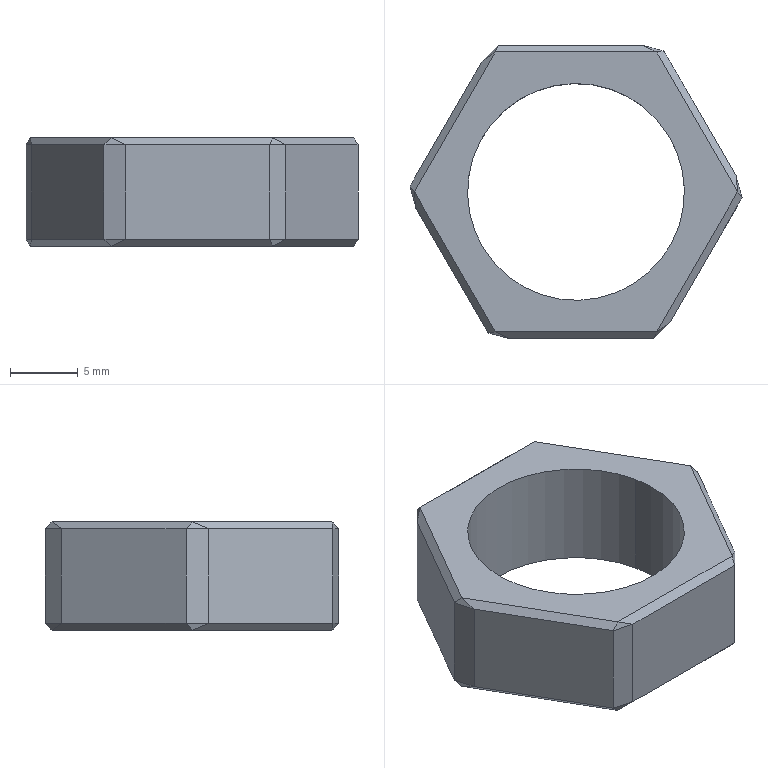Component | SolidWorks | AssemblyVibratoryFeederChassis-1_FootPadScrew-4 | 1 solid | 40 faces | box 24.5 x 21.65 x 8 mm | volume 1608 mm3 | plane 38 | cylinder 2 | commonest cylinder face diameters 16 x2
STEP:
#1=COLOUR_RGB('',0.7922,0.8196,0.9333);
#2=FILL_AREA_STYLE_COLOUR('',#1);
#3=FILL_AREA_STYLE('',(#2));
#4=SURFACE_STYLE_FILL_AREA(#3);
#5=SURFACE_SIDE_STYLE('',(#4));
#6=SURFACE_STYLE_USAGE(.BOTH.,#5);
#7=PRESENTATION_STYLE_ASSIGNMENT((#6));
#8=CARTESIAN_POINT('',(-15.563,9.734,-3.15));
#9=VERTEX_POINT('',#8);
#10=CARTESIAN_POINT('',(-14.945,9.859,-3.15));
#11=VERTEX_POINT('',#10);
#12=CARTESIAN_POINT('',(-15.254,9.796,-3.15));
#13=DIRECTION('',(0.,-0.,1.));
#14=DIRECTION('',(0.98,0.199,0.));
#15=AXIS2_PLACEMENT_3D('',#12,#13,#14);
#16=CIRCLE('',#15,0.315);
#17=EDGE_CURVE('',#9,#11,#16,.T.);
#18=ORIENTED_EDGE('',*,*,#17,.F.);
#19=CARTESIAN_POINT('',(-15.563,9.734,-2.835));
#20=VERTEX_POINT('',#19);
#21=CARTESIAN_POINT('',(-15.563,9.734,-2.835));
#22=DIRECTION('',(0.,-0.,1.));
#23=VECTOR('',#22,39.37);
#24=LINE('',#21,#23);
#25=EDGE_CURVE('',#9,#20,#24,.T.);
#26=ORIENTED_EDGE('',*,*,#25,.T.);
#27=CARTESIAN_POINT('',(-14.945,9.859,-2.835));
#28=VERTEX_POINT('',#27);
#29=CARTESIAN_POINT('',(-15.254,9.796,-2.835));
#30=DIRECTION('',(0.,-0.,1.));
#31=DIRECTION('',(0.98,0.199,0.));
#32=AXIS2_PLACEMENT_3D('',#29,#30,#31);
#33=CIRCLE('',#32,0.315);
#34=EDGE_CURVE('',#20,#28,#33,.T.);
#35=ORIENTED_EDGE('',*,*,#34,.T.);
#36=CARTESIAN_POINT('',(-14.945,9.859,-2.835));
#37=DIRECTION('',(0.,-0.,1.));
#38=VECTOR('',#37,39.37);
#39=LINE('',#36,#38);
#40=EDGE_CURVE('',#11,#28,#39,.T.);
#41=ORIENTED_EDGE('',*,*,#40,.F.);
#42=EDGE_LOOP('',(#18,#26,#35,#41));
#43=FACE_OUTER_BOUND('',#42,.T.);
#44=CARTESIAN_POINT('',(-15.254,9.796,-2.835));
#45=DIRECTION('',(0.,-0.,1.));
#46=DIRECTION('',(0.98,0.199,0.));
#47=AXIS2_PLACEMENT_3D('',#44,#45,#46);
#48=CYLINDRICAL_SURFACE('',#47,0.315);
#49=ADVANCED_FACE('',(#43),#48,.F.);
#50=CARTESIAN_POINT('',(-14.772,9.779,-3.13));
#51=VERTEX_POINT('',#50);
#52=CARTESIAN_POINT('',(-14.772,9.779,-2.854));
#53=VERTEX_POINT('',#52);
#54=CARTESIAN_POINT('',(-14.772,9.779,-2.835));
#55=DIRECTION('',(0.,-0.,1.));
#56=VECTOR('',#55,39.37);
#57=LINE('',#54,#56);
#58=EDGE_CURVE('',#51,#53,#57,.T.);
#59=ORIENTED_EDGE('',*,*,#58,.T.);
#60=CARTESIAN_POINT('',(-14.981,9.417,-2.854));
#61=VERTEX_POINT('',#60);
#62=CARTESIAN_POINT('',(-15.008,9.37,-2.854));
#63=DIRECTION('',(-0.5,-0.866,0.));
#64=VECTOR('',#63,39.37);
#65=LINE('',#62,#64);
#66=EDGE_CURVE('',#53,#61,#65,.T.);
#67=ORIENTED_EDGE('',*,*,#66,.T.);
#68=CARTESIAN_POINT('',(-14.981,9.417,-3.13));
#69=VERTEX_POINT('',#68);
#70=CARTESIAN_POINT('',(-14.981,9.417,-2.835));
#71=DIRECTION('',(-0.,0.,-1.));
#72=VECTOR('',#71,39.37);
#73=LINE('',#70,#72);
#74=EDGE_CURVE('',#61,#69,#73,.T.);
#75=ORIENTED_EDGE('',*,*,#74,.T.);
#76=CARTESIAN_POINT('',(-15.008,9.37,-3.13));
#77=DIRECTION('',(0.5,0.866,-0.));
#78=VECTOR('',#77,39.37);
#79=LINE('',#76,#78);
#80=EDGE_CURVE('',#69,#51,#79,.T.);
#81=ORIENTED_EDGE('',*,*,#80,.T.);
#82=EDGE_LOOP('',(#59,#67,#75,#81));
#83=FACE_OUTER_BOUND('',#82,.T.);
#84=CARTESIAN_POINT('',(-15.008,9.37,-2.835));
#85=DIRECTION('',(-0.866,0.5,0.));
#86=DIRECTION('',(-0.5,-0.866,0.));
#87=AXIS2_PLACEMENT_3D('',#84,#85,#86);
#88=PLANE('',#87);
#89=ADVANCED_FACE('',(#83),#88,.F.);
#90=CARTESIAN_POINT('',(-14.998,10.205,-2.854));
#91=VERTEX_POINT('',#90);
#92=CARTESIAN_POINT('',(-14.789,9.843,-2.854));
#93=VERTEX_POINT('',#92);
#94=CARTESIAN_POINT('',(-14.762,9.796,-2.854));
#95=DIRECTION('',(0.5,-0.866,-0.));
#96=VECTOR('',#95,39.37);
#97=LINE('',#94,#96);
#98=EDGE_CURVE('',#91,#93,#97,.T.);
#99=ORIENTED_EDGE('',*,*,#98,.T.);
#100=CARTESIAN_POINT('',(-14.789,9.843,-3.13));
#101=VERTEX_POINT('',#100);
#102=CARTESIAN_POINT('',(-14.789,9.843,-2.835));
#103=DIRECTION('',(-0.,0.,-1.));
#104=VECTOR('',#103,39.37);
#105=LINE('',#102,#104);
#106=EDGE_CURVE('',#93,#101,#105,.T.);
#107=ORIENTED_EDGE('',*,*,#106,.T.);
#108=CARTESIAN_POINT('',(-14.998,10.205,-3.13));
#109=VERTEX_POINT('',#108);
#110=CARTESIAN_POINT('',(-14.762,9.796,-3.13));
#111=DIRECTION('',(-0.5,0.866,0.));
#112=VECTOR('',#111,39.37);
#113=LINE('',#110,#112);
#114=EDGE_CURVE('',#101,#109,#113,.T.);
#115=ORIENTED_EDGE('',*,*,#114,.T.);
#116=CARTESIAN_POINT('',(-14.998,10.205,-2.835));
#117=DIRECTION('',(0.,-0.,1.));
#118=VECTOR('',#117,39.37);
#119=LINE('',#116,#118);
#120=EDGE_CURVE('',#109,#91,#119,.T.);
#121=ORIENTED_EDGE('',*,*,#120,.T.);
#122=EDGE_LOOP('',(#99,#107,#115,#121));
#123=FACE_OUTER_BOUND('',#122,.T.);
#124=CARTESIAN_POINT('',(-14.762,9.796,-2.835));
#125=DIRECTION('',(-0.866,-0.5,0.));
#126=DIRECTION('',(0.5,-0.866,-0.));
#127=AXIS2_PLACEMENT_3D('',#124,#125,#126);
#128=PLANE('',#127);
#129=ADVANCED_FACE('',(#123),#128,.F.);
#130=CARTESIAN_POINT('',(-15.062,10.222,-3.13));
#131=VERTEX_POINT('',#130);
#132=CARTESIAN_POINT('',(-15.48,10.222,-3.13));
#133=VERTEX_POINT('',#132);
#134=CARTESIAN_POINT('',(-15.008,10.222,-3.13));
#135=DIRECTION('',(-1.,0.,0.));
#136=VECTOR('',#135,39.37);
#137=LINE('',#134,#136);
#138=EDGE_CURVE('',#131,#133,#137,.T.);
#139=ORIENTED_EDGE('',*,*,#138,.T.);
#140=CARTESIAN_POINT('',(-15.48,10.222,-2.854));
#141=VERTEX_POINT('',#140);
#142=CARTESIAN_POINT('',(-15.48,10.222,-2.835));
#143=DIRECTION('',(0.,-0.,1.));
#144=VECTOR('',#143,39.37);
#145=LINE('',#142,#144);
#146=EDGE_CURVE('',#133,#141,#145,.T.);
#147=ORIENTED_EDGE('',*,*,#146,.T.);
#148=CARTESIAN_POINT('',(-15.062,10.222,-2.854));
#149=VERTEX_POINT('',#148);
#150=CARTESIAN_POINT('',(-15.008,10.222,-2.854));
#151=DIRECTION('',(1.,-0.,-0.));
#152=VECTOR('',#151,39.37);
#153=LINE('',#150,#152);
#154=EDGE_CURVE('',#141,#149,#153,.T.);
#155=ORIENTED_EDGE('',*,*,#154,.T.);
#156=CARTESIAN_POINT('',(-15.062,10.222,-2.835));
#157=DIRECTION('',(-0.,0.,-1.));
#158=VECTOR('',#157,39.37);
#159=LINE('',#156,#158);
#160=EDGE_CURVE('',#149,#131,#159,.T.);
#161=ORIENTED_EDGE('',*,*,#160,.T.);
#162=EDGE_LOOP('',(#139,#147,#155,#161));
#163=FACE_OUTER_BOUND('',#162,.T.);
#164=CARTESIAN_POINT('',(-15.008,10.222,-2.835));
#165=DIRECTION('',(-0.,-1.,-0.));
#166=DIRECTION('',(1.,-0.,-0.));
#167=AXIS2_PLACEMENT_3D('',#164,#165,#166);
#168=PLANE('',#167);
#169=ADVANCED_FACE('',(#163),#168,.F.);
#170=CARTESIAN_POINT('',(-15.736,9.813,-3.13));
#171=VERTEX_POINT('',#170);
#172=CARTESIAN_POINT('',(-15.736,9.813,-2.854));
#173=VERTEX_POINT('',#172);
#174=CARTESIAN_POINT('',(-15.736,9.813,-2.835));
#175=DIRECTION('',(0.,-0.,1.));
#176=VECTOR('',#175,39.37);
#177=LINE('',#174,#176);
#178=EDGE_CURVE('',#171,#173,#177,.T.);
#179=ORIENTED_EDGE('',*,*,#178,.T.);
#180=CARTESIAN_POINT('',(-15.527,10.176,-2.854));
#181=VERTEX_POINT('',#180);
#182=CARTESIAN_POINT('',(-15.5,10.222,-2.854));
#183=DIRECTION('',(0.5,0.866,-0.));
#184=VECTOR('',#183,39.37);
#185=LINE('',#182,#184);
#186=EDGE_CURVE('',#173,#181,#185,.T.);
#187=ORIENTED_EDGE('',*,*,#186,.T.);
#188=CARTESIAN_POINT('',(-15.527,10.176,-3.13));
#189=VERTEX_POINT('',#188);
#190=CARTESIAN_POINT('',(-15.527,10.176,-2.835));
#191=DIRECTION('',(-0.,0.,-1.));
#192=VECTOR('',#191,39.37);
#193=LINE('',#190,#192);
#194=EDGE_CURVE('',#181,#189,#193,.T.);
#195=ORIENTED_EDGE('',*,*,#194,.T.);
#196=CARTESIAN_POINT('',(-15.5,10.222,-3.13));
#197=DIRECTION('',(-0.5,-0.866,0.));
#198=VECTOR('',#197,39.37);
#199=LINE('',#196,#198);
#200=EDGE_CURVE('',#189,#171,#199,.T.);
#201=ORIENTED_EDGE('',*,*,#200,.T.);
#202=EDGE_LOOP('',(#179,#187,#195,#201));
#203=FACE_OUTER_BOUND('',#202,.T.);
#204=CARTESIAN_POINT('',(-15.5,10.222,-2.835));
#205=DIRECTION('',(0.866,-0.5,-0.));
#206=DIRECTION('',(0.5,0.866,-0.));
#207=AXIS2_PLACEMENT_3D('',#204,#205,#206);
#208=PLANE('',#207);
#209=ADVANCED_FACE('',(#203),#208,.F.);
#210=CARTESIAN_POINT('',(-15.51,9.387,-3.13));
#211=VERTEX_POINT('',#210);
#212=CARTESIAN_POINT('',(-15.51,9.387,-2.854));
#213=VERTEX_POINT('',#212);
#214=CARTESIAN_POINT('',(-15.51,9.387,-2.835));
#215=DIRECTION('',(0.,-0.,1.));
#216=VECTOR('',#215,39.37);
#217=LINE('',#214,#216);
#218=EDGE_CURVE('',#211,#213,#217,.T.);
#219=ORIENTED_EDGE('',*,*,#218,.T.);
#220=CARTESIAN_POINT('',(-15.719,9.75,-2.854));
#221=VERTEX_POINT('',#220);
#222=CARTESIAN_POINT('',(-15.746,9.796,-2.854));
#223=DIRECTION('',(-0.5,0.866,0.));
#224=VECTOR('',#223,39.37);
#225=LINE('',#222,#224);
#226=EDGE_CURVE('',#213,#221,#225,.T.);
#227=ORIENTED_EDGE('',*,*,#226,.T.);
#228=CARTESIAN_POINT('',(-15.719,9.75,-3.13));
#229=VERTEX_POINT('',#228);
#230=CARTESIAN_POINT('',(-15.719,9.75,-2.835));
#231=DIRECTION('',(-0.,0.,-1.));
#232=VECTOR('',#231,39.37);
#233=LINE('',#230,#232);
#234=EDGE_CURVE('',#221,#229,#233,.T.);
#235=ORIENTED_EDGE('',*,*,#234,.T.);
#236=CARTESIAN_POINT('',(-15.746,9.796,-3.13));
#237=DIRECTION('',(0.5,-0.866,-0.));
#238=VECTOR('',#237,39.37);
#239=LINE('',#236,#238);
#240=EDGE_CURVE('',#229,#211,#239,.T.);
#241=ORIENTED_EDGE('',*,*,#240,.T.);
#242=EDGE_LOOP('',(#219,#227,#235,#241));
#243=FACE_OUTER_BOUND('',#242,.T.);
#244=CARTESIAN_POINT('',(-15.746,9.796,-2.835));
#245=DIRECTION('',(0.866,0.5,-0.));
#246=DIRECTION('',(-0.5,0.866,0.));
#247=AXIS2_PLACEMENT_3D('',#244,#245,#246);
#248=PLANE('',#247);
#249=ADVANCED_FACE('',(#243),#248,.F.);
#250=CARTESIAN_POINT('',(-15.028,9.37,-3.13));
#251=VERTEX_POINT('',#250);
#252=CARTESIAN_POINT('',(-15.028,9.37,-2.854));
#253=VERTEX_POINT('',#252);
#254=CARTESIAN_POINT('',(-15.028,9.37,-2.835));
#255=DIRECTION('',(0.,-0.,1.));
#256=VECTOR('',#255,39.37);
#257=LINE('',#254,#256);
#258=EDGE_CURVE('',#251,#253,#257,.T.);
#259=ORIENTED_EDGE('',*,*,#258,.T.);
#260=CARTESIAN_POINT('',(-15.446,9.37,-2.854));
#261=VERTEX_POINT('',#260);
#262=CARTESIAN_POINT('',(-15.5,9.37,-2.854));
#263=DIRECTION('',(-1.,0.,0.));
#264=VECTOR('',#263,39.37);
#265=LINE('',#262,#264);
#266=EDGE_CURVE('',#253,#261,#265,.T.);
#267=ORIENTED_EDGE('',*,*,#266,.T.);
#268=CARTESIAN_POINT('',(-15.446,9.37,-3.13));
#269=VERTEX_POINT('',#268);
#270=CARTESIAN_POINT('',(-15.446,9.37,-2.835));
#271=DIRECTION('',(-0.,0.,-1.));
#272=VECTOR('',#271,39.37);
#273=LINE('',#270,#272);
#274=EDGE_CURVE('',#261,#269,#273,.T.);
#275=ORIENTED_EDGE('',*,*,#274,.T.);
#276=CARTESIAN_POINT('',(-15.5,9.37,-3.13));
#277=DIRECTION('',(1.,-0.,-0.));
#278=VECTOR('',#277,39.37);
#279=LINE('',#276,#278);
#280=EDGE_CURVE('',#269,#251,#279,.T.);
#281=ORIENTED_EDGE('',*,*,#280,.T.);
#282=EDGE_LOOP('',(#259,#267,#275,#281));
#283=FACE_OUTER_BOUND('',#282,.T.);
#284=CARTESIAN_POINT('',(-15.5,9.37,-2.835));
#285=DIRECTION('',(0.,1.,0.));
#286=DIRECTION('',(-1.,0.,0.));
#287=AXIS2_PLACEMENT_3D('',#284,#285,#286);
#288=PLANE('',#287);
#289=ADVANCED_FACE('',(#283),#288,.F.);
#290=CARTESIAN_POINT('',(-15.489,9.39,-2.835));
#291=VERTEX_POINT('',#290);
#292=CARTESIAN_POINT('',(-15.019,9.39,-2.835));
#293=VERTEX_POINT('',#292);
#294=CARTESIAN_POINT('',(-15.008,9.39,-2.835));
#295=DIRECTION('',(1.,-0.,-0.));
#296=VECTOR('',#295,39.37);
#297=LINE('',#294,#296);
#298=EDGE_CURVE('',#291,#293,#297,.T.);
#299=ORIENTED_EDGE('',*,*,#298,.T.);
#300=CARTESIAN_POINT('',(-14.784,9.796,-2.835));
#301=VERTEX_POINT('',#300);
#302=CARTESIAN_POINT('',(-14.779,9.806,-2.835));
#303=DIRECTION('',(0.5,0.866,-0.));
#304=VECTOR('',#303,39.37);
#305=LINE('',#302,#304);
#306=EDGE_CURVE('',#293,#301,#305,.T.);
#307=ORIENTED_EDGE('',*,*,#306,.T.);
#308=CARTESIAN_POINT('',(-15.019,10.203,-2.835));
#309=VERTEX_POINT('',#308);
#310=CARTESIAN_POINT('',(-15.025,10.213,-2.835));
#311=DIRECTION('',(-0.5,0.866,0.));
#312=VECTOR('',#311,39.37);
#313=LINE('',#310,#312);
#314=EDGE_CURVE('',#301,#309,#313,.T.);
#315=ORIENTED_EDGE('',*,*,#314,.T.);
#316=CARTESIAN_POINT('',(-15.489,10.203,-2.835));
#317=VERTEX_POINT('',#316);
#318=CARTESIAN_POINT('',(-15.5,10.203,-2.835));
#319=DIRECTION('',(-1.,0.,0.));
#320=VECTOR('',#319,39.37);
#321=LINE('',#318,#320);
#322=EDGE_CURVE('',#309,#317,#321,.T.);
#323=ORIENTED_EDGE('',*,*,#322,.T.);
#324=CARTESIAN_POINT('',(-15.723,9.796,-2.835));
#325=VERTEX_POINT('',#324);
#326=CARTESIAN_POINT('',(-15.729,9.786,-2.835));
#327=DIRECTION('',(-0.5,-0.866,0.));
#328=VECTOR('',#327,39.37);
#329=LINE('',#326,#328);
#330=EDGE_CURVE('',#317,#325,#329,.T.);
#331=ORIENTED_EDGE('',*,*,#330,.T.);
#332=CARTESIAN_POINT('',(-15.483,9.38,-2.835));
#333=DIRECTION('',(0.5,-0.866,-0.));
#334=VECTOR('',#333,39.37);
#335=LINE('',#332,#334);
#336=EDGE_CURVE('',#325,#291,#335,.T.);
#337=ORIENTED_EDGE('',*,*,#336,.T.);
#338=EDGE_LOOP('',(#299,#307,#315,#323,#331,#337));
#339=FACE_OUTER_BOUND('',#338,.T.);
#340=CARTESIAN_POINT('',(-15.254,9.796,-2.835));
#341=DIRECTION('',(0.,-0.,1.));
#342=DIRECTION('',(0.98,0.199,0.));
#343=AXIS2_PLACEMENT_3D('',#340,#341,#342);
#344=CIRCLE('',#343,0.315);
#345=EDGE_CURVE('',#28,#20,#344,.T.);
#346=ORIENTED_EDGE('',*,*,#345,.F.);
#347=ORIENTED_EDGE('',*,*,#34,.F.);
#348=EDGE_LOOP('',(#346,#347));
#349=FACE_BOUND('',#348,.T.);
#350=CARTESIAN_POINT('',(-14.762,9.796,-2.835));
#351=DIRECTION('',(0.,-0.,1.));
#352=DIRECTION('',(0.98,0.199,-0.));
#353=AXIS2_PLACEMENT_3D('',#350,#351,#352);
#354=PLANE('',#353);
#355=ADVANCED_FACE('',(#339,#349),#354,.T.);
#356=CARTESIAN_POINT('',(-15.019,10.203,-3.15));
#357=VERTEX_POINT('',#356);
#358=CARTESIAN_POINT('',(-14.784,9.796,-3.15));
#359=VERTEX_POINT('',#358);
#360=CARTESIAN_POINT('',(-14.779,9.786,-3.15));
#361=DIRECTION('',(0.5,-0.866,-0.));
#362=VECTOR('',#361,39.37);
#363=LINE('',#360,#362);
#364=EDGE_CURVE('',#357,#359,#363,.T.);
#365=ORIENTED_EDGE('',*,*,#364,.T.);
#366=CARTESIAN_POINT('',(-15.019,9.39,-3.15));
#367=VERTEX_POINT('',#366);
#368=CARTESIAN_POINT('',(-14.779,9.806,-3.15));
#369=DIRECTION('',(-0.5,-0.866,0.));
#370=VECTOR('',#369,39.37);
#371=LINE('',#368,#370);
#372=EDGE_CURVE('',#359,#367,#371,.T.);
#373=ORIENTED_EDGE('',*,*,#372,.T.);
#374=CARTESIAN_POINT('',(-15.489,9.39,-3.15));
#375=VERTEX_POINT('',#374);
#376=CARTESIAN_POINT('',(-14.762,9.39,-3.15));
#377=DIRECTION('',(-1.,0.,0.));
#378=VECTOR('',#377,39.37);
#379=LINE('',#376,#378);
#380=EDGE_CURVE('',#367,#375,#379,.T.);
#381=ORIENTED_EDGE('',*,*,#380,.T.);
#382=CARTESIAN_POINT('',(-15.723,9.796,-3.15));
#383=VERTEX_POINT('',#382);
#384=CARTESIAN_POINT('',(-15.483,9.38,-3.15));
#385=DIRECTION('',(-0.5,0.866,0.));
#386=VECTOR('',#385,39.37);
#387=LINE('',#384,#386);
#388=EDGE_CURVE('',#375,#383,#387,.T.);
#389=ORIENTED_EDGE('',*,*,#388,.T.);
#390=CARTESIAN_POINT('',(-15.489,10.203,-3.15));
#391=VERTEX_POINT('',#390);
#392=CARTESIAN_POINT('',(-15.483,10.213,-3.15));
#393=DIRECTION('',(0.5,0.866,-0.));
#394=VECTOR('',#393,39.37);
#395=LINE('',#392,#394);
#396=EDGE_CURVE('',#383,#391,#395,.T.);
#397=ORIENTED_EDGE('',*,*,#396,.T.);
#398=CARTESIAN_POINT('',(-14.762,10.203,-3.15));
#399=DIRECTION('',(1.,-0.,-0.));
#400=VECTOR('',#399,39.37);
#401=LINE('',#398,#400);
#402=EDGE_CURVE('',#391,#357,#401,.T.);
#403=ORIENTED_EDGE('',*,*,#402,.T.);
#404=EDGE_LOOP('',(#365,#373,#381,#389,#397,#403));
#405=FACE_OUTER_BOUND('',#404,.T.);
#406=CARTESIAN_POINT('',(-15.254,9.796,-3.15));
#407=DIRECTION('',(0.,-0.,1.));
#408=DIRECTION('',(0.98,0.199,0.));
#409=AXIS2_PLACEMENT_3D('',#406,#407,#408);
#410=CIRCLE('',#409,0.315);
#411=EDGE_CURVE('',#11,#9,#410,.T.);
#412=ORIENTED_EDGE('',*,*,#411,.T.);
#413=ORIENTED_EDGE('',*,*,#17,.T.);
#414=EDGE_LOOP('',(#412,#413));
#415=FACE_BOUND('',#414,.T.);
#416=CARTESIAN_POINT('',(-14.762,9.796,-3.15));
#417=DIRECTION('',(0.,-0.,1.));
#418=DIRECTION('',(0.98,0.199,-0.));
#419=AXIS2_PLACEMENT_3D('',#416,#417,#418);
#420=PLANE('',#419);
#421=ADVANCED_FACE('',(#405,#415),#420,.F.);
#422=ORIENTED_EDGE('',*,*,#25,.F.);
#423=ORIENTED_EDGE('',*,*,#411,.F.);
#424=ORIENTED_EDGE('',*,*,#40,.T.);
#425=ORIENTED_EDGE('',*,*,#345,.T.);
#426=EDGE_LOOP('',(#422,#423,#424,#425));
#427=FACE_OUTER_BOUND('',#426,.T.);
#428=CARTESIAN_POINT('',(-15.254,9.796,-2.835));
#429=DIRECTION('',(0.,-0.,1.));
#430=DIRECTION('',(0.98,0.199,0.));
#431=AXIS2_PLACEMENT_3D('',#428,#429,#430);
#432=CYLINDRICAL_SURFACE('',#431,0.315);
#433=ADVANCED_FACE('',(#427),#432,.F.);
#434=CARTESIAN_POINT('',(-15.48,10.222,-2.854));
#435=DIRECTION('',(-0.7071,-0.7071,0.));
#436=VECTOR('',#435,39.37);
#437=LINE('',#434,#436);
#438=EDGE_CURVE('',#141,#181,#437,.T.);
#439=ORIENTED_EDGE('',*,*,#438,.F.);
#440=ORIENTED_EDGE('',*,*,#146,.F.);
#441=CARTESIAN_POINT('',(-15.527,10.176,-3.13));
#442=DIRECTION('',(0.7071,0.7071,0.));
#443=VECTOR('',#442,39.37);
#444=LINE('',#441,#443);
#445=EDGE_CURVE('',#189,#133,#444,.T.);
#446=ORIENTED_EDGE('',*,*,#445,.F.);
#447=ORIENTED_EDGE('',*,*,#194,.F.);
#448=EDGE_LOOP('',(#439,#440,#446,#447));
#449=FACE_OUTER_BOUND('',#448,.T.);
#450=CARTESIAN_POINT('',(-15.527,10.176,-2.835));
#451=DIRECTION('',(0.7071,-0.7071,-0.));
#452=DIRECTION('',(0.7071,0.7071,-0.));
#453=AXIS2_PLACEMENT_3D('',#450,#451,#452);
#454=PLANE('',#453);
#455=ADVANCED_FACE('',(#449),#454,.F.);
#456=CARTESIAN_POINT('',(-15.48,10.222,-2.854));
#457=DIRECTION('',(-0.2863,-0.6775,0.6775));
#458=VECTOR('',#457,39.37);
#459=LINE('',#456,#458);
#460=EDGE_CURVE('',#141,#317,#459,.T.);
#461=ORIENTED_EDGE('',*,*,#460,.F.);
#462=ORIENTED_EDGE('',*,*,#438,.T.);
#463=CARTESIAN_POINT('',(-15.482,10.208,-2.831));
#464=DIRECTION('',(-0.754,-0.53,-0.388));
#465=VECTOR('',#464,39.37);
#466=LINE('',#463,#465);
#467=EDGE_CURVE('',#317,#181,#466,.T.);
#468=ORIENTED_EDGE('',*,*,#467,.F.);
#469=EDGE_LOOP('',(#461,#462,#468));
#470=FACE_OUTER_BOUND('',#469,.T.);
#471=CARTESIAN_POINT('',(-15.48,10.222,-2.854));
#472=DIRECTION('',(-0.6547,0.6547,0.378));
#473=DIRECTION('',(-0.7071,-0.7071,0.));
#474=AXIS2_PLACEMENT_3D('',#471,#472,#473);
#475=PLANE('',#474);
#476=ADVANCED_FACE('',(#470),#475,.T.);
#477=CARTESIAN_POINT('',(-15.527,10.176,-3.13));
#478=DIRECTION('',(0.754,0.53,-0.388));
#479=VECTOR('',#478,39.37);
#480=LINE('',#477,#479);
#481=EDGE_CURVE('',#189,#391,#480,.T.);
#482=ORIENTED_EDGE('',*,*,#481,.F.);
#483=ORIENTED_EDGE('',*,*,#445,.T.);
#484=CARTESIAN_POINT('',(-15.493,10.192,-3.16));
#485=DIRECTION('',(0.2863,0.6775,0.6775));
#486=VECTOR('',#485,39.37);
#487=LINE('',#484,#486);
#488=EDGE_CURVE('',#391,#133,#487,.T.);
#489=ORIENTED_EDGE('',*,*,#488,.F.);
#490=EDGE_LOOP('',(#482,#483,#489));
#491=FACE_OUTER_BOUND('',#490,.T.);
#492=CARTESIAN_POINT('',(-15.527,10.176,-3.13));
#493=DIRECTION('',(-0.6547,0.6547,-0.378));
#494=DIRECTION('',(-0.7071,-0.7071,0.));
#495=AXIS2_PLACEMENT_3D('',#492,#493,#494);
#496=PLANE('',#495);
#497=ADVANCED_FACE('',(#491),#496,.T.);
#498=ORIENTED_EDGE('',*,*,#467,.T.);
#499=ORIENTED_EDGE('',*,*,#186,.F.);
#500=CARTESIAN_POINT('',(-15.736,9.813,-2.854));
#501=DIRECTION('',(-0.4436,0.5867,-0.6775));
#502=VECTOR('',#501,39.37);
#503=LINE('',#500,#502);
#504=EDGE_CURVE('',#325,#173,#503,.T.);
#505=ORIENTED_EDGE('',*,*,#504,.F.);
#506=ORIENTED_EDGE('',*,*,#330,.F.);
#507=EDGE_LOOP('',(#498,#499,#505,#506));
#508=FACE_OUTER_BOUND('',#507,.T.);
#509=CARTESIAN_POINT('',(-15.483,10.213,-2.835));
#510=DIRECTION('',(-0.6124,0.3536,0.7071));
#511=DIRECTION('',(0.7843,0.1593,0.5996));
#512=AXIS2_PLACEMENT_3D('',#509,#510,#511);
#513=PLANE('',#512);
#514=ADVANCED_FACE('',(#508),#513,.T.);
#515=ORIENTED_EDGE('',*,*,#460,.T.);
#516=ORIENTED_EDGE('',*,*,#322,.F.);
#517=CARTESIAN_POINT('',(-15.062,10.222,-2.854));
#518=DIRECTION('',(0.836,-0.388,0.388));
#519=VECTOR('',#518,39.37);
#520=LINE('',#517,#519);
#521=EDGE_CURVE('',#149,#309,#520,.T.);
#522=ORIENTED_EDGE('',*,*,#521,.F.);
#523=ORIENTED_EDGE('',*,*,#154,.F.);
#524=EDGE_LOOP('',(#515,#516,#522,#523));
#525=FACE_OUTER_BOUND('',#524,.T.);
#526=CARTESIAN_POINT('',(-14.762,10.203,-2.835));
#527=DIRECTION('',(0.,0.7071,0.7071));
#528=DIRECTION('',(0.1422,-0.6999,0.6999));
#529=AXIS2_PLACEMENT_3D('',#526,#527,#528);
#530=PLANE('',#529);
#531=ADVANCED_FACE('',(#525),#530,.T.);
#532=CARTESIAN_POINT('',(-15.062,10.222,-3.13));
#533=DIRECTION('',(0.9659,-0.2588,0.));
#534=VECTOR('',#533,39.37);
#535=LINE('',#532,#534);
#536=EDGE_CURVE('',#131,#109,#535,.T.);
#537=ORIENTED_EDGE('',*,*,#536,.F.);
#538=ORIENTED_EDGE('',*,*,#160,.F.);
#539=CARTESIAN_POINT('',(-15.062,10.222,-2.854));
#540=DIRECTION('',(-0.9659,0.2588,0.));
#541=VECTOR('',#540,39.37);
#542=LINE('',#539,#541);
#543=EDGE_CURVE('',#91,#149,#542,.T.);
#544=ORIENTED_EDGE('',*,*,#543,.F.);
#545=ORIENTED_EDGE('',*,*,#120,.F.);
#546=EDGE_LOOP('',(#537,#538,#544,#545));
#547=FACE_OUTER_BOUND('',#546,.T.);
#548=CARTESIAN_POINT('',(-15.062,10.222,-2.835));
#549=DIRECTION('',(-0.2588,-0.9659,-0.));
#550=DIRECTION('',(0.9659,-0.2588,-0.));
#551=AXIS2_PLACEMENT_3D('',#548,#549,#550);
#552=PLANE('',#551);
#553=ADVANCED_FACE('',(#547),#552,.F.);
#554=ORIENTED_EDGE('',*,*,#488,.T.);
#555=ORIENTED_EDGE('',*,*,#138,.F.);
#556=CARTESIAN_POINT('',(-15.062,10.222,-3.13));
#557=DIRECTION('',(-0.836,0.388,0.388));
#558=VECTOR('',#557,39.37);
#559=LINE('',#556,#558);
#560=EDGE_CURVE('',#357,#131,#559,.T.);
#561=ORIENTED_EDGE('',*,*,#560,.F.);
#562=ORIENTED_EDGE('',*,*,#402,.F.);
#563=EDGE_LOOP('',(#554,#555,#561,#562));
#564=FACE_OUTER_BOUND('',#563,.T.);
#565=CARTESIAN_POINT('',(-15.008,10.222,-3.13));
#566=DIRECTION('',(-0.,-0.7071,0.7071));
#567=DIRECTION('',(0.1422,-0.6999,-0.6999));
#568=AXIS2_PLACEMENT_3D('',#565,#566,#567);
#569=PLANE('',#568);
#570=ADVANCED_FACE('',(#564),#569,.F.);
#571=ORIENTED_EDGE('',*,*,#481,.T.);
#572=ORIENTED_EDGE('',*,*,#396,.F.);
#573=CARTESIAN_POINT('',(-15.716,9.787,-3.16));
#574=DIRECTION('',(0.4436,-0.5867,-0.6775));
#575=VECTOR('',#574,39.37);
#576=LINE('',#573,#575);
#577=EDGE_CURVE('',#171,#383,#576,.T.);
#578=ORIENTED_EDGE('',*,*,#577,.F.);
#579=ORIENTED_EDGE('',*,*,#200,.F.);
#580=EDGE_LOOP('',(#571,#572,#578,#579));
#581=FACE_OUTER_BOUND('',#580,.T.);
#582=CARTESIAN_POINT('',(-15.5,10.222,-3.13));
#583=DIRECTION('',(0.6124,-0.3536,0.7071));
#584=DIRECTION('',(0.7843,0.1593,-0.5996));
#585=AXIS2_PLACEMENT_3D('',#582,#583,#584);
#586=PLANE('',#585);
#587=ADVANCED_FACE('',(#581),#586,.F.);
#588=CARTESIAN_POINT('',(-15.736,9.813,-2.854));
#589=DIRECTION('',(0.2588,-0.9659,0.));
#590=VECTOR('',#589,39.37);
#591=LINE('',#588,#590);
#592=EDGE_CURVE('',#173,#221,#591,.T.);
#593=ORIENTED_EDGE('',*,*,#592,.F.);
#594=ORIENTED_EDGE('',*,*,#178,.F.);
#595=CARTESIAN_POINT('',(-15.719,9.75,-3.13));
#596=DIRECTION('',(-0.2588,0.9659,-0.));
#597=VECTOR('',#596,39.37);
#598=LINE('',#595,#597);
#599=EDGE_CURVE('',#229,#171,#598,.T.);
#600=ORIENTED_EDGE('',*,*,#599,.F.);
#601=ORIENTED_EDGE('',*,*,#234,.F.);
#602=EDGE_LOOP('',(#593,#594,#600,#601));
#603=FACE_OUTER_BOUND('',#602,.T.);
#604=CARTESIAN_POINT('',(-15.719,9.75,-2.835));
#605=DIRECTION('',(0.9659,0.2588,-0.));
#606=DIRECTION('',(-0.2588,0.9659,0.));
#607=AXIS2_PLACEMENT_3D('',#604,#605,#606);
#608=PLANE('',#607);
#609=ADVANCED_FACE('',(#603),#608,.F.);
#610=ORIENTED_EDGE('',*,*,#504,.T.);
#611=ORIENTED_EDGE('',*,*,#592,.T.);
#612=CARTESIAN_POINT('',(-15.724,9.805,-2.831));
#613=DIRECTION('',(0.08199,-0.918,-0.388));
#614=VECTOR('',#613,39.37);
#615=LINE('',#612,#614);
#616=EDGE_CURVE('',#325,#221,#615,.T.);
#617=ORIENTED_EDGE('',*,*,#616,.F.);
#618=EDGE_LOOP('',(#610,#611,#617));
#619=FACE_OUTER_BOUND('',#618,.T.);
#620=CARTESIAN_POINT('',(-15.736,9.813,-2.854));
#621=DIRECTION('',(-0.8943,-0.2396,0.378));
#622=DIRECTION('',(0.371,0.07535,0.9256));
#623=AXIS2_PLACEMENT_3D('',#620,#621,#622);
#624=PLANE('',#623);
#625=ADVANCED_FACE('',(#619),#624,.T.);
#626=ORIENTED_EDGE('',*,*,#543,.T.);
#627=ORIENTED_EDGE('',*,*,#521,.T.);
#628=CARTESIAN_POINT('',(-15.031,10.201,-2.824));
#629=DIRECTION('',(-0.7299,-0.09077,0.6775));
#630=VECTOR('',#629,39.37);
#631=LINE('',#628,#630);
#632=EDGE_CURVE('',#91,#309,#631,.T.);
#633=ORIENTED_EDGE('',*,*,#632,.F.);
#634=EDGE_LOOP('',(#626,#627,#633));
#635=FACE_OUTER_BOUND('',#634,.T.);
#636=CARTESIAN_POINT('',(-15.062,10.222,-2.854));
#637=DIRECTION('',(0.2396,0.8943,0.378));
#638=DIRECTION('',(-0.9659,0.2588,0.));
#639=AXIS2_PLACEMENT_3D('',#636,#637,#638);
#640=PLANE('',#639);
#641=ADVANCED_FACE('',(#635),#640,.T.);
#642=ORIENTED_EDGE('',*,*,#560,.T.);
#643=ORIENTED_EDGE('',*,*,#536,.T.);
#644=CARTESIAN_POINT('',(-15.031,10.201,-3.16));
#645=DIRECTION('',(0.7299,0.09077,0.6775));
#646=VECTOR('',#645,39.37);
#647=LINE('',#644,#646);
#648=EDGE_CURVE('',#357,#109,#647,.T.);
#649=ORIENTED_EDGE('',*,*,#648,.F.);
#650=EDGE_LOOP('',(#642,#643,#649));
#651=FACE_OUTER_BOUND('',#650,.T.);
#652=CARTESIAN_POINT('',(-15.062,10.222,-3.13));
#653=DIRECTION('',(0.2396,0.8943,-0.378));
#654=DIRECTION('',(-0.9659,0.2588,0.));
#655=AXIS2_PLACEMENT_3D('',#652,#653,#654);
#656=PLANE('',#655);
#657=ADVANCED_FACE('',(#651),#656,.T.);
#658=ORIENTED_EDGE('',*,*,#599,.T.);
#659=ORIENTED_EDGE('',*,*,#577,.T.);
#660=CARTESIAN_POINT('',(-15.719,9.75,-3.13));
#661=DIRECTION('',(-0.08199,0.918,-0.388));
#662=VECTOR('',#661,39.37);
#663=LINE('',#660,#662);
#664=EDGE_CURVE('',#229,#383,#663,.T.);
#665=ORIENTED_EDGE('',*,*,#664,.F.);
#666=EDGE_LOOP('',(#658,#659,#665));
#667=FACE_OUTER_BOUND('',#666,.T.);
#668=CARTESIAN_POINT('',(-15.719,9.75,-3.13));
#669=DIRECTION('',(-0.8943,-0.2396,-0.378));
#670=DIRECTION('',(-0.371,-0.07535,0.9256));
#671=AXIS2_PLACEMENT_3D('',#668,#669,#670);
#672=PLANE('',#671);
#673=ADVANCED_FACE('',(#667),#672,.T.);
#674=ORIENTED_EDGE('',*,*,#616,.T.);
#675=ORIENTED_EDGE('',*,*,#226,.F.);
#676=CARTESIAN_POINT('',(-15.51,9.387,-2.854));
#677=DIRECTION('',(-0.7299,-0.09077,-0.6775));
#678=VECTOR('',#677,39.37);
#679=LINE('',#676,#678);
#680=EDGE_CURVE('',#291,#213,#679,.T.);
#681=ORIENTED_EDGE('',*,*,#680,.F.);
#682=ORIENTED_EDGE('',*,*,#336,.F.);
#683=EDGE_LOOP('',(#674,#675,#681,#682));
#684=FACE_OUTER_BOUND('',#683,.T.);
#685=CARTESIAN_POINT('',(-15.483,9.38,-2.835));
#686=DIRECTION('',(-0.6124,-0.3536,0.7071));
#687=DIRECTION('',(0.7111,0.1444,0.6881));
#688=AXIS2_PLACEMENT_3D('',#685,#686,#687);
#689=PLANE('',#688);
#690=ADVANCED_FACE('',(#684),#689,.T.);
#691=ORIENTED_EDGE('',*,*,#632,.T.);
#692=ORIENTED_EDGE('',*,*,#314,.F.);
#693=CARTESIAN_POINT('',(-14.784,9.788,-2.831));
#694=DIRECTION('',(0.08199,-0.918,0.388));
#695=VECTOR('',#694,39.37);
#696=LINE('',#693,#695);
#697=EDGE_CURVE('',#93,#301,#696,.T.);
#698=ORIENTED_EDGE('',*,*,#697,.F.);
#699=ORIENTED_EDGE('',*,*,#98,.F.);
#700=EDGE_LOOP('',(#691,#692,#698,#699));
#701=FACE_OUTER_BOUND('',#700,.T.);
#702=CARTESIAN_POINT('',(-14.779,9.786,-2.835));
#703=DIRECTION('',(0.6124,0.3536,0.7071));
#704=DIRECTION('',(0.7111,0.1444,-0.6881));
#705=AXIS2_PLACEMENT_3D('',#702,#703,#704);
#706=PLANE('',#705);
#707=ADVANCED_FACE('',(#701),#706,.T.);
#708=CARTESIAN_POINT('',(-14.789,9.843,-3.13));
#709=DIRECTION('',(0.2588,-0.9659,-0.));
#710=VECTOR('',#709,39.37);
#711=LINE('',#708,#710);
#712=EDGE_CURVE('',#101,#51,#711,.T.);
#713=ORIENTED_EDGE('',*,*,#712,.F.);
#714=ORIENTED_EDGE('',*,*,#106,.F.);
#715=CARTESIAN_POINT('',(-14.772,9.779,-2.854));
#716=DIRECTION('',(-0.2588,0.9659,0.));
#717=VECTOR('',#716,39.37);
#718=LINE('',#715,#717);
#719=EDGE_CURVE('',#53,#93,#718,.T.);
#720=ORIENTED_EDGE('',*,*,#719,.F.);
#721=ORIENTED_EDGE('',*,*,#58,.F.);
#722=EDGE_LOOP('',(#713,#714,#720,#721));
#723=FACE_OUTER_BOUND('',#722,.T.);
#724=CARTESIAN_POINT('',(-14.789,9.843,-2.835));
#725=DIRECTION('',(-0.9659,-0.2588,0.));
#726=DIRECTION('',(0.2588,-0.9659,-0.));
#727=AXIS2_PLACEMENT_3D('',#724,#725,#726);
#728=PLANE('',#727);
#729=ADVANCED_FACE('',(#723),#728,.F.);
#730=ORIENTED_EDGE('',*,*,#648,.T.);
#731=ORIENTED_EDGE('',*,*,#114,.F.);
#732=CARTESIAN_POINT('',(-14.789,9.843,-3.13));
#733=DIRECTION('',(-0.08199,0.918,0.388));
#734=VECTOR('',#733,39.37);
#735=LINE('',#732,#734);
#736=EDGE_CURVE('',#359,#101,#735,.T.);
#737=ORIENTED_EDGE('',*,*,#736,.F.);
#738=ORIENTED_EDGE('',*,*,#364,.F.);
#739=EDGE_LOOP('',(#730,#731,#737,#738));
#740=FACE_OUTER_BOUND('',#739,.T.);
#741=CARTESIAN_POINT('',(-14.762,9.796,-3.13));
#742=DIRECTION('',(-0.6124,-0.3536,0.7071));
#743=DIRECTION('',(0.7111,0.1444,0.6881));
#744=AXIS2_PLACEMENT_3D('',#741,#742,#743);
#745=PLANE('',#744);
#746=ADVANCED_FACE('',(#740),#745,.F.);
#747=ORIENTED_EDGE('',*,*,#664,.T.);
#748=ORIENTED_EDGE('',*,*,#388,.F.);
#749=CARTESIAN_POINT('',(-15.477,9.391,-3.16));
#750=DIRECTION('',(0.7299,0.09077,-0.6775));
#751=VECTOR('',#750,39.37);
#752=LINE('',#749,#751);
#753=EDGE_CURVE('',#211,#375,#752,.T.);
#754=ORIENTED_EDGE('',*,*,#753,.F.);
#755=ORIENTED_EDGE('',*,*,#240,.F.);
#756=EDGE_LOOP('',(#747,#748,#754,#755));
#757=FACE_OUTER_BOUND('',#756,.T.);
#758=CARTESIAN_POINT('',(-15.746,9.796,-3.13));
#759=DIRECTION('',(0.6124,0.3536,0.7071));
#760=DIRECTION('',(0.7111,0.1444,-0.6881));
#761=AXIS2_PLACEMENT_3D('',#758,#759,#760);
#762=PLANE('',#761);
#763=ADVANCED_FACE('',(#757),#762,.F.);
#764=CARTESIAN_POINT('',(-15.51,9.387,-2.854));
#765=DIRECTION('',(0.9659,-0.2588,-0.));
#766=VECTOR('',#765,39.37);
#767=LINE('',#764,#766);
#768=EDGE_CURVE('',#213,#261,#767,.T.);
#769=ORIENTED_EDGE('',*,*,#768,.F.);
#770=ORIENTED_EDGE('',*,*,#218,.F.);
#771=CARTESIAN_POINT('',(-15.446,9.37,-3.13));
#772=DIRECTION('',(-0.9659,0.2588,-0.));
#773=VECTOR('',#772,39.37);
#774=LINE('',#771,#773);
#775=EDGE_CURVE('',#269,#211,#774,.T.);
#776=ORIENTED_EDGE('',*,*,#775,.F.);
#777=ORIENTED_EDGE('',*,*,#274,.F.);
#778=EDGE_LOOP('',(#769,#770,#776,#777));
#779=FACE_OUTER_BOUND('',#778,.T.);
#780=CARTESIAN_POINT('',(-15.446,9.37,-2.835));
#781=DIRECTION('',(0.2588,0.9659,0.));
#782=DIRECTION('',(-0.9659,0.2588,0.));
#783=AXIS2_PLACEMENT_3D('',#780,#781,#782);
#784=PLANE('',#783);
#785=ADVANCED_FACE('',(#779),#784,.F.);
#786=ORIENTED_EDGE('',*,*,#680,.T.);
#787=ORIENTED_EDGE('',*,*,#768,.T.);
#788=CARTESIAN_POINT('',(-15.496,9.393,-2.831));
#789=DIRECTION('',(0.836,-0.388,-0.388));
#790=VECTOR('',#789,39.37);
#791=LINE('',#788,#790);
#792=EDGE_CURVE('',#291,#261,#791,.T.);
#793=ORIENTED_EDGE('',*,*,#792,.F.);
#794=EDGE_LOOP('',(#786,#787,#793));
#795=FACE_OUTER_BOUND('',#794,.T.);
#796=CARTESIAN_POINT('',(-15.51,9.387,-2.854));
#797=DIRECTION('',(-0.2396,-0.8943,0.378));
#798=DIRECTION('',(0.9659,-0.2588,-0.));
#799=AXIS2_PLACEMENT_3D('',#796,#797,#798);
#800=PLANE('',#799);
#801=ADVANCED_FACE('',(#795),#800,.T.);
#802=ORIENTED_EDGE('',*,*,#719,.T.);
#803=ORIENTED_EDGE('',*,*,#697,.T.);
#804=CARTESIAN_POINT('',(-14.772,9.779,-2.854));
#805=DIRECTION('',(-0.4436,0.5867,0.6775));
#806=VECTOR('',#805,39.37);
#807=LINE('',#804,#806);
#808=EDGE_CURVE('',#53,#301,#807,.T.);
#809=ORIENTED_EDGE('',*,*,#808,.F.);
#810=EDGE_LOOP('',(#802,#803,#809));
#811=FACE_OUTER_BOUND('',#810,.T.);
#812=CARTESIAN_POINT('',(-14.772,9.779,-2.854));
#813=DIRECTION('',(0.8943,0.2396,0.378));
#814=DIRECTION('',(0.371,0.07535,-0.9256));
#815=AXIS2_PLACEMENT_3D('',#812,#813,#814);
#816=PLANE('',#815);
#817=ADVANCED_FACE('',(#811),#816,.T.);
#818=ORIENTED_EDGE('',*,*,#736,.T.);
#819=ORIENTED_EDGE('',*,*,#712,.T.);
#820=CARTESIAN_POINT('',(-14.792,9.806,-3.16));
#821=DIRECTION('',(0.4436,-0.5867,0.6775));
#822=VECTOR('',#821,39.37);
#823=LINE('',#820,#822);
#824=EDGE_CURVE('',#359,#51,#823,.T.);
#825=ORIENTED_EDGE('',*,*,#824,.F.);
#826=EDGE_LOOP('',(#818,#819,#825));
#827=FACE_OUTER_BOUND('',#826,.T.);
#828=CARTESIAN_POINT('',(-14.789,9.843,-3.13));
#829=DIRECTION('',(0.8943,0.2396,-0.378));
#830=DIRECTION('',(-0.371,-0.07535,-0.9256));
#831=AXIS2_PLACEMENT_3D('',#828,#829,#830);
#832=PLANE('',#831);
#833=ADVANCED_FACE('',(#827),#832,.T.);
#834=ORIENTED_EDGE('',*,*,#775,.T.);
#835=ORIENTED_EDGE('',*,*,#753,.T.);
#836=CARTESIAN_POINT('',(-15.446,9.37,-3.13));
#837=DIRECTION('',(-0.836,0.388,-0.388));
#838=VECTOR('',#837,39.37);
#839=LINE('',#836,#838);
#840=EDGE_CURVE('',#269,#375,#839,.T.);
#841=ORIENTED_EDGE('',*,*,#840,.F.);
#842=EDGE_LOOP('',(#834,#835,#841));
#843=FACE_OUTER_BOUND('',#842,.T.);
#844=CARTESIAN_POINT('',(-15.446,9.37,-3.13));
#845=DIRECTION('',(-0.2396,-0.8943,-0.378));
#846=DIRECTION('',(0.9659,-0.2588,-0.));
#847=AXIS2_PLACEMENT_3D('',#844,#845,#846);
#848=PLANE('',#847);
#849=ADVANCED_FACE('',(#843),#848,.T.);
#850=ORIENTED_EDGE('',*,*,#792,.T.);
#851=ORIENTED_EDGE('',*,*,#266,.F.);
#852=CARTESIAN_POINT('',(-15.028,9.37,-2.854));
#853=DIRECTION('',(-0.2863,-0.6775,-0.6775));
#854=VECTOR('',#853,39.37);
#855=LINE('',#852,#854);
#856=EDGE_CURVE('',#293,#253,#855,.T.);
#857=ORIENTED_EDGE('',*,*,#856,.F.);
#858=ORIENTED_EDGE('',*,*,#298,.F.);
#859=EDGE_LOOP('',(#850,#851,#857,#858));
#860=FACE_OUTER_BOUND('',#859,.T.);
#861=CARTESIAN_POINT('',(-14.762,9.39,-2.835));
#862=DIRECTION('',(-0.,-0.7071,0.7071));
#863=DIRECTION('',(0.1422,-0.6999,-0.6999));
#864=AXIS2_PLACEMENT_3D('',#861,#862,#863);
#865=PLANE('',#864);
#866=ADVANCED_FACE('',(#860),#865,.T.);
#867=ORIENTED_EDGE('',*,*,#808,.T.);
#868=ORIENTED_EDGE('',*,*,#306,.F.);
#869=CARTESIAN_POINT('',(-15.026,9.385,-2.831));
#870=DIRECTION('',(-0.754,-0.53,0.388));
#871=VECTOR('',#870,39.37);
#872=LINE('',#869,#871);
#873=EDGE_CURVE('',#61,#293,#872,.T.);
#874=ORIENTED_EDGE('',*,*,#873,.F.);
#875=ORIENTED_EDGE('',*,*,#66,.F.);
#876=EDGE_LOOP('',(#867,#868,#874,#875));
#877=FACE_OUTER_BOUND('',#876,.T.);
#878=CARTESIAN_POINT('',(-14.779,9.806,-2.835));
#879=DIRECTION('',(0.6124,-0.3536,0.7071));
#880=DIRECTION('',(0.7843,0.1593,-0.5996));
#881=AXIS2_PLACEMENT_3D('',#878,#879,#880);
#882=PLANE('',#881);
#883=ADVANCED_FACE('',(#877),#882,.T.);
#884=ORIENTED_EDGE('',*,*,#824,.T.);
#885=ORIENTED_EDGE('',*,*,#80,.F.);
#886=CARTESIAN_POINT('',(-14.981,9.417,-3.13));
#887=DIRECTION('',(0.754,0.53,0.388));
#888=VECTOR('',#887,39.37);
#889=LINE('',#886,#888);
#890=EDGE_CURVE('',#367,#69,#889,.T.);
#891=ORIENTED_EDGE('',*,*,#890,.F.);
#892=ORIENTED_EDGE('',*,*,#372,.F.);
#893=EDGE_LOOP('',(#884,#885,#891,#892));
#894=FACE_OUTER_BOUND('',#893,.T.);
#895=CARTESIAN_POINT('',(-15.008,9.37,-3.13));
#896=DIRECTION('',(-0.6124,0.3536,0.7071));
#897=DIRECTION('',(0.7843,0.1593,0.5996));
#898=AXIS2_PLACEMENT_3D('',#895,#896,#897);
#899=PLANE('',#898);
#900=ADVANCED_FACE('',(#894),#899,.F.);
#901=ORIENTED_EDGE('',*,*,#840,.T.);
#902=ORIENTED_EDGE('',*,*,#380,.F.);
#903=CARTESIAN_POINT('',(-15.015,9.4,-3.16));
#904=DIRECTION('',(0.2863,0.6775,-0.6775));
#905=VECTOR('',#904,39.37);
#906=LINE('',#903,#905);
#907=EDGE_CURVE('',#251,#367,#906,.T.);
#908=ORIENTED_EDGE('',*,*,#907,.F.);
#909=ORIENTED_EDGE('',*,*,#280,.F.);
#910=EDGE_LOOP('',(#901,#902,#908,#909));
#911=FACE_OUTER_BOUND('',#910,.T.);
#912=CARTESIAN_POINT('',(-15.5,9.37,-3.13));
#913=DIRECTION('',(0.,0.7071,0.7071));
#914=DIRECTION('',(0.1422,-0.6999,0.6999));
#915=AXIS2_PLACEMENT_3D('',#912,#913,#914);
#916=PLANE('',#915);
#917=ADVANCED_FACE('',(#911),#916,.F.);
#918=ORIENTED_EDGE('',*,*,#873,.T.);
#919=ORIENTED_EDGE('',*,*,#856,.T.);
#920=CARTESIAN_POINT('',(-15.028,9.37,-2.854));
#921=DIRECTION('',(-0.7071,-0.7071,0.));
#922=VECTOR('',#921,39.37);
#923=LINE('',#920,#922);
#924=EDGE_CURVE('',#61,#253,#923,.T.);
#925=ORIENTED_EDGE('',*,*,#924,.F.);
#926=EDGE_LOOP('',(#918,#919,#925));
#927=FACE_OUTER_BOUND('',#926,.T.);
#928=CARTESIAN_POINT('',(-15.028,9.37,-2.854));
#929=DIRECTION('',(0.6547,-0.6547,0.378));
#930=DIRECTION('',(0.7071,0.7071,-0.));
#931=AXIS2_PLACEMENT_3D('',#928,#929,#930);
#932=PLANE('',#931);
#933=ADVANCED_FACE('',(#927),#932,.T.);
#934=ORIENTED_EDGE('',*,*,#907,.T.);
#935=ORIENTED_EDGE('',*,*,#890,.T.);
#936=CARTESIAN_POINT('',(-14.981,9.417,-3.13));
#937=DIRECTION('',(0.7071,0.7071,-0.));
#938=VECTOR('',#937,39.37);
#939=LINE('',#936,#938);
#940=EDGE_CURVE('',#251,#69,#939,.T.);
#941=ORIENTED_EDGE('',*,*,#940,.F.);
#942=EDGE_LOOP('',(#934,#935,#941));
#943=FACE_OUTER_BOUND('',#942,.T.);
#944=CARTESIAN_POINT('',(-14.981,9.417,-3.13));
#945=DIRECTION('',(0.6547,-0.6547,-0.378));
#946=DIRECTION('',(0.7071,0.7071,-0.));
#947=AXIS2_PLACEMENT_3D('',#944,#945,#946);
#948=PLANE('',#947);
#949=ADVANCED_FACE('',(#943),#948,.T.);
#950=ORIENTED_EDGE('',*,*,#924,.T.);
#951=ORIENTED_EDGE('',*,*,#258,.F.);
#952=ORIENTED_EDGE('',*,*,#940,.T.);
#953=ORIENTED_EDGE('',*,*,#74,.F.);
#954=EDGE_LOOP('',(#950,#951,#952,#953));
#955=FACE_OUTER_BOUND('',#954,.T.);
#956=CARTESIAN_POINT('',(-14.981,9.417,-2.835));
#957=DIRECTION('',(-0.7071,0.7071,0.));
#958=DIRECTION('',(-0.7071,-0.7071,0.));
#959=AXIS2_PLACEMENT_3D('',#956,#957,#958);
#960=PLANE('',#959);
#961=ADVANCED_FACE('',(#955),#960,.F.);
#962=CLOSED_SHELL('',(#49,#89,#129,#169,#209,#249,#289,#355,#421,#433,#455,#476,#497,#514,#531,#553,#570,#587,#609,#625,#641,#657,#673,#690,#707,#729,#746,#763,#785,#801,#817,#833,#849,#866,#883,#900,#917,#933,#949,#961));
#963=MANIFOLD_SOLID_BREP('',#962);
#964=STYLED_ITEM('',(#7),#963);
#965=(LENGTH_UNIT()NAMED_UNIT(*)SI_UNIT($,.METRE.));
#966=LENGTH_MEASURE_WITH_UNIT(LENGTH_MEASURE(0.0254),#965);
#967=DIMENSIONAL_EXPONENTS(1.,0.,0.,0.,0.,0.,0.);
#968=(CONVERSION_BASED_UNIT('',#966)LENGTH_UNIT()NAMED_UNIT(#967));
#969=UNCERTAINTY_MEASURE_WITH_UNIT(LENGTH_MEASURE(0.00001),#968,'','');
#970=(NAMED_UNIT(*)PLANE_ANGLE_UNIT()SI_UNIT($,.RADIAN.));
#971=(NAMED_UNIT(*)SI_UNIT($,.STERADIAN.)SOLID_ANGLE_UNIT());
#972=(GEOMETRIC_REPRESENTATION_CONTEXT(3)GLOBAL_UNCERTAINTY_ASSIGNED_CONTEXT((#969))GLOBAL_UNIT_ASSIGNED_CONTEXT((#968,#970,#971))REPRESENTATION_CONTEXT('',''));
#973=MECHANICAL_DESIGN_GEOMETRIC_PRESENTATION_REPRESENTATION('',(#964),#972);
#974=PRESENTATION_LAYER_ASSIGNMENT('','',(#964));
#975=CARTESIAN_POINT('',(0.,0.,0.));
#976=DIRECTION('',(0.,0.,1.));
#977=DIRECTION('',(1.,0.,0.));
#978=AXIS2_PLACEMENT_3D('',#975,#976,#977);
#979=(LENGTH_UNIT()NAMED_UNIT(*)SI_UNIT($,.METRE.));
#980=LENGTH_MEASURE_WITH_UNIT(LENGTH_MEASURE(0.0254),#979);
#981=DIMENSIONAL_EXPONENTS(1.,0.,0.,0.,0.,0.,0.);
#982=(CONVERSION_BASED_UNIT('',#980)LENGTH_UNIT()NAMED_UNIT(#981));
#983=UNCERTAINTY_MEASURE_WITH_UNIT(LENGTH_MEASURE(0.00001),#982,'','');
#984=(NAMED_UNIT(*)PLANE_ANGLE_UNIT()SI_UNIT($,.RADIAN.));
#985=(NAMED_UNIT(*)SI_UNIT($,.STERADIAN.)SOLID_ANGLE_UNIT());
#986=(GEOMETRIC_REPRESENTATION_CONTEXT(3)GLOBAL_UNCERTAINTY_ASSIGNED_CONTEXT((#983))GLOBAL_UNIT_ASSIGNED_CONTEXT((#982,#984,#985))REPRESENTATION_CONTEXT('',''));
#987=ADVANCED_BREP_SHAPE_REPRESENTATION('',(#963,#978),#986);